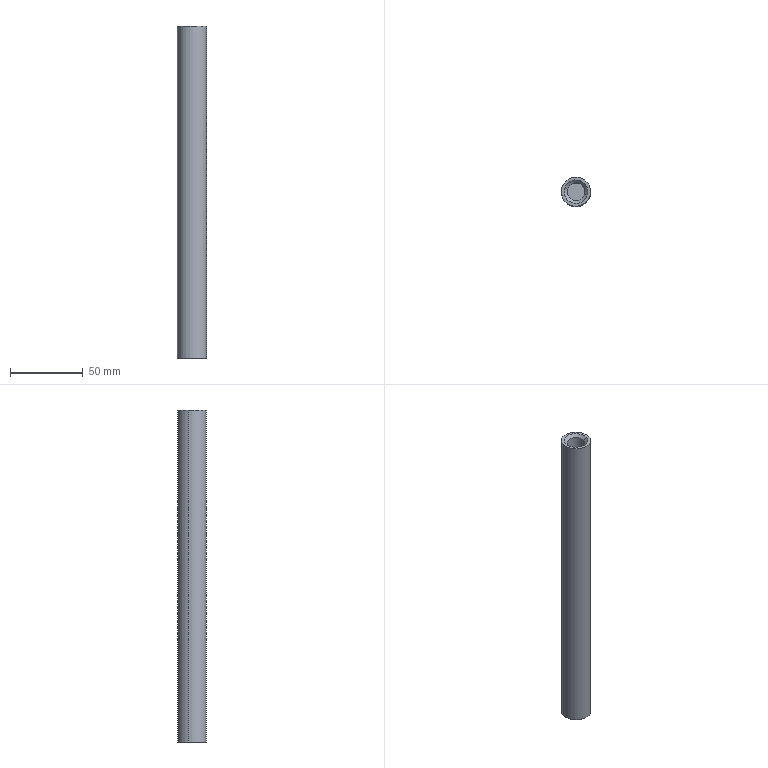Component | SolidWorks | BearingPressPartN-1 | 1 solid | 13 faces | box 20 x 20 x 228 mm | volume 58262 mm3 | cylinder 6 | cone 4 | plane 3 | commonest cylinder face diameters 14.5 x2 12.2 x2 20 x2
build123d program:
from build123d import *

# Parameters (mm, degrees)
SKETCH1_R                  = 10
BOSS_EXTRUDE1_DEPTH        = 228
SKETCH2_R                  = 6.1
CUT_EXTRUDE1_DEPTH         = 60
CHAMFER1_SIZE              = 2
M16X1_5_TAPPED_HOLE1_D     = 14.5
M16X1_5_TAPPED_HOLE1_DEPTH = 36.5
M16X1_5_TAPPED_HOLE1_TIP   = 4.356


with BuildPart() as part:
    # Sketch1 → Boss-Extrude1 (new body)
    with BuildSketch(Plane.XY):
        with Locations(Location((0, 0, 0), (0, 0, 180))):
            Circle(SKETCH1_R)
    extrude(amount=BOSS_EXTRUDE1_DEPTH)

    # Sketch2 → Cut-Extrude1 (cut)
    with BuildSketch(Plane(origin=(0, 0, 0), x_dir=(-1, 0, 0), z_dir=(0, 0, -1))):
        Circle(SKETCH2_R)
    extrude(amount=-CUT_EXTRUDE1_DEPTH, mode=Mode.SUBTRACT)

    # Chamfer1
    chamfer1_edges = [part.edges().sort_by_distance(p)[0] for p in [
        (6.1, 0, 0),
    ]]
    chamfer(chamfer1_edges, length=CHAMFER1_SIZE)

    # M16x1.5 Tapped Hole1
    with Locations(Plane.XY.offset(228)):
        with Locations((0, 0)):
            Hole(M16X1_5_TAPPED_HOLE1_D / 2, depth=M16X1_5_TAPPED_HOLE1_DEPTH)
            with Locations((0, 0, -(M16X1_5_TAPPED_HOLE1_DEPTH + M16X1_5_TAPPED_HOLE1_TIP / 2))):  # 118° drill point
                Cone(0, M16X1_5_TAPPED_HOLE1_D / 2, M16X1_5_TAPPED_HOLE1_TIP, mode=Mode.SUBTRACT)


solid = part.part

# Placed as in the assembly
solid = solid.moved(Location((447.676, 127.964, -266.218), (180, 0, 0)))
STEP:
#1=COLOUR_RGB('',0.7922,0.8196,0.9333);
#2=FILL_AREA_STYLE_COLOUR('',#1);
#3=FILL_AREA_STYLE('',(#2));
#4=SURFACE_STYLE_FILL_AREA(#3);
#5=SURFACE_SIDE_STYLE('',(#4));
#6=SURFACE_STYLE_USAGE(.BOTH.,#5);
#7=PRESENTATION_STYLE_ASSIGNMENT((#6));
#8=CARTESIAN_POINT('',(17.35,5.114,-18.02));
#9=VERTEX_POINT('',#8);
#10=CARTESIAN_POINT('',(17.9,4.962,-18.02));
#11=VERTEX_POINT('',#10);
#12=CARTESIAN_POINT('',(17.625,5.038,-18.02));
#13=DIRECTION('',(0.,-0.,-1.));
#14=DIRECTION('',(0.9638,-0.2665,0.));
#15=AXIS2_PLACEMENT_3D('',#12,#13,#14);
#16=CIRCLE('',#15,0.2854);
#17=EDGE_CURVE('',#9,#11,#16,.T.);
#18=ORIENTED_EDGE('',*,*,#17,.F.);
#19=CARTESIAN_POINT('',(17.35,5.114,-19.457));
#20=VERTEX_POINT('',#19);
#21=CARTESIAN_POINT('',(17.35,5.114,-19.457));
#22=DIRECTION('',(0.,-0.,-1.));
#23=VECTOR('',#22,39.37);
#24=LINE('',#21,#23);
#25=EDGE_CURVE('',#9,#20,#24,.T.);
#26=ORIENTED_EDGE('',*,*,#25,.T.);
#27=CARTESIAN_POINT('',(17.9,4.962,-19.457));
#28=VERTEX_POINT('',#27);
#29=CARTESIAN_POINT('',(17.625,5.038,-19.457));
#30=DIRECTION('',(0.,-0.,-1.));
#31=DIRECTION('',(0.9638,-0.2665,0.));
#32=AXIS2_PLACEMENT_3D('',#29,#30,#31);
#33=CIRCLE('',#32,0.2854);
#34=EDGE_CURVE('',#20,#28,#33,.T.);
#35=ORIENTED_EDGE('',*,*,#34,.T.);
#36=CARTESIAN_POINT('',(17.9,4.962,-19.457));
#37=DIRECTION('',(0.,-0.,-1.));
#38=VECTOR('',#37,39.37);
#39=LINE('',#36,#38);
#40=EDGE_CURVE('',#11,#28,#39,.T.);
#41=ORIENTED_EDGE('',*,*,#40,.F.);
#42=EDGE_LOOP('',(#18,#26,#35,#41));
#43=FACE_OUTER_BOUND('',#42,.T.);
#44=CARTESIAN_POINT('',(17.625,5.038,-19.457));
#45=DIRECTION('',(0.,-0.,-1.));
#46=DIRECTION('',(0.9638,-0.2665,0.));
#47=AXIS2_PLACEMENT_3D('',#44,#45,#46);
#48=CYLINDRICAL_SURFACE('',#47,0.2854);
#49=ADVANCED_FACE('',(#43),#48,.F.);
#50=CARTESIAN_POINT('',(17.625,5.038,-17.849));
#51=VERTEX_POINT('',#50);
#52=CARTESIAN_POINT('',(17.9,4.962,-18.02));
#53=DIRECTION('',(0.8262,-0.2284,-0.515));
#54=VECTOR('',#53,39.37);
#55=LINE('',#52,#54);
#56=EDGE_CURVE('',#51,#11,#55,.T.);
#57=ORIENTED_EDGE('',*,*,#56,.F.);
#58=CARTESIAN_POINT('',(17.35,5.114,-18.02));
#59=DIRECTION('',(-0.8262,0.2284,-0.515));
#60=VECTOR('',#59,39.37);
#61=LINE('',#58,#60);
#62=EDGE_CURVE('',#51,#9,#61,.T.);
#63=ORIENTED_EDGE('',*,*,#62,.T.);
#64=ORIENTED_EDGE('',*,*,#17,.T.);
#65=EDGE_LOOP('',(#57,#63,#64));
#66=FACE_OUTER_BOUND('',#65,.T.);
#67=CARTESIAN_POINT('',(17.625,5.038,-18.02));
#68=DIRECTION('',(0.,-0.,-1.));
#69=DIRECTION('',(0.9638,-0.2665,0.));
#70=AXIS2_PLACEMENT_3D('',#67,#68,#69);
#71=CONICAL_SURFACE('',#70,0.2854,1.03);
#72=ADVANCED_FACE('',(#66),#71,.F.);
#73=CARTESIAN_POINT('',(17.857,4.974,-10.56));
#74=VERTEX_POINT('',#73);
#75=CARTESIAN_POINT('',(17.394,5.102,-10.56));
#76=VERTEX_POINT('',#75);
#77=CARTESIAN_POINT('',(17.625,5.038,-10.56));
#78=DIRECTION('',(-0.,0.,1.));
#79=DIRECTION('',(0.9638,-0.2665,0.));
#80=AXIS2_PLACEMENT_3D('',#77,#78,#79);
#81=CIRCLE('',#80,0.2402);
#82=EDGE_CURVE('',#74,#76,#81,.T.);
#83=ORIENTED_EDGE('',*,*,#82,.F.);
#84=CARTESIAN_POINT('',(17.932,4.953,-10.481));
#85=VERTEX_POINT('',#84);
#86=CARTESIAN_POINT('',(17.857,4.974,-10.56));
#87=DIRECTION('',(0.6815,-0.1884,0.7071));
#88=VECTOR('',#87,39.37);
#89=LINE('',#86,#88);
#90=EDGE_CURVE('',#74,#85,#89,.T.);
#91=ORIENTED_EDGE('',*,*,#90,.T.);
#92=CARTESIAN_POINT('',(17.318,5.123,-10.481));
#93=VERTEX_POINT('',#92);
#94=CARTESIAN_POINT('',(17.625,5.038,-10.481));
#95=DIRECTION('',(0.,-0.,-1.));
#96=DIRECTION('',(0.9638,-0.2665,0.));
#97=AXIS2_PLACEMENT_3D('',#94,#95,#96);
#98=CIRCLE('',#97,0.3189);
#99=EDGE_CURVE('',#93,#85,#98,.T.);
#100=ORIENTED_EDGE('',*,*,#99,.F.);
#101=CARTESIAN_POINT('',(17.394,5.102,-10.56));
#102=DIRECTION('',(-0.6815,0.1884,0.7071));
#103=VECTOR('',#102,39.37);
#104=LINE('',#101,#103);
#105=EDGE_CURVE('',#76,#93,#104,.T.);
#106=ORIENTED_EDGE('',*,*,#105,.F.);
#107=EDGE_LOOP('',(#83,#91,#100,#106));
#108=FACE_OUTER_BOUND('',#107,.T.);
#109=CARTESIAN_POINT('',(17.625,5.038,-10.56));
#110=DIRECTION('',(-0.,0.,1.));
#111=DIRECTION('',(-0.9638,0.2665,0.));
#112=AXIS2_PLACEMENT_3D('',#109,#110,#111);
#113=CONICAL_SURFACE('',#112,0.2402,0.7854);
#114=ADVANCED_FACE('',(#108),#113,.F.);
#115=CARTESIAN_POINT('',(17.857,4.974,-12.843));
#116=VERTEX_POINT('',#115);
#117=CARTESIAN_POINT('',(17.394,5.102,-12.843));
#118=VERTEX_POINT('',#117);
#119=CARTESIAN_POINT('',(17.625,5.038,-12.843));
#120=DIRECTION('',(-0.,0.,1.));
#121=DIRECTION('',(-0.9638,0.2665,0.));
#122=AXIS2_PLACEMENT_3D('',#119,#120,#121);
#123=CIRCLE('',#122,0.2402);
#124=EDGE_CURVE('',#116,#118,#123,.T.);
#125=ORIENTED_EDGE('',*,*,#124,.F.);
#126=CARTESIAN_POINT('',(17.857,4.974,-12.843));
#127=DIRECTION('',(-0.,0.,1.));
#128=VECTOR('',#127,39.37);
#129=LINE('',#126,#128);
#130=EDGE_CURVE('',#116,#74,#129,.T.);
#131=ORIENTED_EDGE('',*,*,#130,.T.);
#132=ORIENTED_EDGE('',*,*,#82,.T.);
#133=CARTESIAN_POINT('',(17.394,5.102,-12.843));
#134=DIRECTION('',(-0.,0.,1.));
#135=VECTOR('',#134,39.37);
#136=LINE('',#133,#135);
#137=EDGE_CURVE('',#118,#76,#136,.T.);
#138=ORIENTED_EDGE('',*,*,#137,.F.);
#139=EDGE_LOOP('',(#125,#131,#132,#138));
#140=FACE_OUTER_BOUND('',#139,.T.);
#141=CARTESIAN_POINT('',(17.625,5.038,-12.843));
#142=DIRECTION('',(-0.,0.,1.));
#143=DIRECTION('',(-0.9638,0.2665,0.));
#144=AXIS2_PLACEMENT_3D('',#141,#142,#143);
#145=CYLINDRICAL_SURFACE('',#144,0.2402);
#146=ADVANCED_FACE('',(#140),#145,.F.);
#147=CARTESIAN_POINT('',(18.005,4.933,-19.457));
#148=VERTEX_POINT('',#147);
#149=CARTESIAN_POINT('',(17.246,5.143,-19.457));
#150=VERTEX_POINT('',#149);
#151=CARTESIAN_POINT('',(17.625,5.038,-19.457));
#152=DIRECTION('',(0.,-0.,-1.));
#153=DIRECTION('',(0.9638,-0.2665,0.));
#154=AXIS2_PLACEMENT_3D('',#151,#152,#153);
#155=CIRCLE('',#154,0.3937);
#156=EDGE_CURVE('',#148,#150,#155,.T.);
#157=ORIENTED_EDGE('',*,*,#156,.F.);
#158=CARTESIAN_POINT('',(18.005,4.933,-10.481));
#159=VERTEX_POINT('',#158);
#160=CARTESIAN_POINT('',(18.005,4.933,-19.457));
#161=DIRECTION('',(-0.,0.,1.));
#162=VECTOR('',#161,39.37);
#163=LINE('',#160,#162);
#164=EDGE_CURVE('',#148,#159,#163,.T.);
#165=ORIENTED_EDGE('',*,*,#164,.T.);
#166=CARTESIAN_POINT('',(17.246,5.143,-10.481));
#167=VERTEX_POINT('',#166);
#168=CARTESIAN_POINT('',(17.625,5.038,-10.481));
#169=DIRECTION('',(0.,-0.,-1.));
#170=DIRECTION('',(0.9638,-0.2665,0.));
#171=AXIS2_PLACEMENT_3D('',#168,#169,#170);
#172=CIRCLE('',#171,0.3937);
#173=EDGE_CURVE('',#159,#167,#172,.T.);
#174=ORIENTED_EDGE('',*,*,#173,.T.);
#175=CARTESIAN_POINT('',(17.246,5.143,-19.457));
#176=DIRECTION('',(-0.,0.,1.));
#177=VECTOR('',#176,39.37);
#178=LINE('',#175,#177);
#179=EDGE_CURVE('',#150,#167,#178,.T.);
#180=ORIENTED_EDGE('',*,*,#179,.F.);
#181=EDGE_LOOP('',(#157,#165,#174,#180));
#182=FACE_OUTER_BOUND('',#181,.T.);
#183=CARTESIAN_POINT('',(17.625,5.038,-19.457));
#184=DIRECTION('',(-0.,0.,1.));
#185=DIRECTION('',(-0.9638,0.2665,0.));
#186=AXIS2_PLACEMENT_3D('',#183,#184,#185);
#187=CYLINDRICAL_SURFACE('',#186,0.3937);
#188=ADVANCED_FACE('',(#182),#187,.T.);
#189=ORIENTED_EDGE('',*,*,#164,.F.);
#190=CARTESIAN_POINT('',(17.625,5.038,-19.457));
#191=DIRECTION('',(0.,-0.,-1.));
#192=DIRECTION('',(0.9638,-0.2665,0.));
#193=AXIS2_PLACEMENT_3D('',#190,#191,#192);
#194=CIRCLE('',#193,0.3937);
#195=EDGE_CURVE('',#150,#148,#194,.T.);
#196=ORIENTED_EDGE('',*,*,#195,.F.);
#197=ORIENTED_EDGE('',*,*,#179,.T.);
#198=CARTESIAN_POINT('',(17.625,5.038,-10.481));
#199=DIRECTION('',(0.,-0.,-1.));
#200=DIRECTION('',(0.9638,-0.2665,0.));
#201=AXIS2_PLACEMENT_3D('',#198,#199,#200);
#202=CIRCLE('',#201,0.3937);
#203=EDGE_CURVE('',#167,#159,#202,.T.);
#204=ORIENTED_EDGE('',*,*,#203,.T.);
#205=EDGE_LOOP('',(#189,#196,#197,#204));
#206=FACE_OUTER_BOUND('',#205,.T.);
#207=CARTESIAN_POINT('',(17.625,5.038,-19.457));
#208=DIRECTION('',(-0.,0.,1.));
#209=DIRECTION('',(-0.9638,0.2665,0.));
#210=AXIS2_PLACEMENT_3D('',#207,#208,#209);
#211=CYLINDRICAL_SURFACE('',#210,0.3937);
#212=ADVANCED_FACE('',(#206),#211,.T.);
#213=CARTESIAN_POINT('',(17.625,5.038,-19.457));
#214=DIRECTION('',(0.,-0.,-1.));
#215=DIRECTION('',(0.9638,-0.2665,0.));
#216=AXIS2_PLACEMENT_3D('',#213,#214,#215);
#217=CIRCLE('',#216,0.2854);
#218=EDGE_CURVE('',#28,#20,#217,.T.);
#219=ORIENTED_EDGE('',*,*,#218,.F.);
#220=ORIENTED_EDGE('',*,*,#34,.F.);
#221=EDGE_LOOP('',(#219,#220));
#222=FACE_BOUND('',#221,.T.);
#223=ORIENTED_EDGE('',*,*,#195,.T.);
#224=ORIENTED_EDGE('',*,*,#156,.T.);
#225=EDGE_LOOP('',(#223,#224));
#226=FACE_OUTER_BOUND('',#225,.T.);
#227=CARTESIAN_POINT('',(17.625,5.038,-19.457));
#228=DIRECTION('',(0.,-0.,-1.));
#229=DIRECTION('',(0.9638,-0.2665,0.));
#230=AXIS2_PLACEMENT_3D('',#227,#228,#229);
#231=PLANE('',#230);
#232=ADVANCED_FACE('',(#222,#226),#231,.T.);
#233=ORIENTED_EDGE('',*,*,#99,.T.);
#234=CARTESIAN_POINT('',(17.625,5.038,-10.481));
#235=DIRECTION('',(0.,-0.,-1.));
#236=DIRECTION('',(0.9638,-0.2665,0.));
#237=AXIS2_PLACEMENT_3D('',#234,#235,#236);
#238=CIRCLE('',#237,0.3189);
#239=EDGE_CURVE('',#85,#93,#238,.T.);
#240=ORIENTED_EDGE('',*,*,#239,.T.);
#241=EDGE_LOOP('',(#233,#240));
#242=FACE_BOUND('',#241,.T.);
#243=ORIENTED_EDGE('',*,*,#203,.F.);
#244=ORIENTED_EDGE('',*,*,#173,.F.);
#245=EDGE_LOOP('',(#243,#244));
#246=FACE_OUTER_BOUND('',#245,.T.);
#247=CARTESIAN_POINT('',(17.625,5.038,-10.481));
#248=DIRECTION('',(0.,-0.,-1.));
#249=DIRECTION('',(0.9638,-0.2665,0.));
#250=AXIS2_PLACEMENT_3D('',#247,#248,#249);
#251=PLANE('',#250);
#252=ADVANCED_FACE('',(#242,#246),#251,.F.);
#253=ORIENTED_EDGE('',*,*,#130,.F.);
#254=CARTESIAN_POINT('',(17.625,5.038,-12.843));
#255=DIRECTION('',(-0.,0.,1.));
#256=DIRECTION('',(-0.9638,0.2665,0.));
#257=AXIS2_PLACEMENT_3D('',#254,#255,#256);
#258=CIRCLE('',#257,0.2402);
#259=EDGE_CURVE('',#118,#116,#258,.T.);
#260=ORIENTED_EDGE('',*,*,#259,.F.);
#261=ORIENTED_EDGE('',*,*,#137,.T.);
#262=CARTESIAN_POINT('',(17.625,5.038,-10.56));
#263=DIRECTION('',(-0.,0.,1.));
#264=DIRECTION('',(0.9638,-0.2665,0.));
#265=AXIS2_PLACEMENT_3D('',#262,#263,#264);
#266=CIRCLE('',#265,0.2402);
#267=EDGE_CURVE('',#76,#74,#266,.T.);
#268=ORIENTED_EDGE('',*,*,#267,.T.);
#269=EDGE_LOOP('',(#253,#260,#261,#268));
#270=FACE_OUTER_BOUND('',#269,.T.);
#271=CARTESIAN_POINT('',(17.625,5.038,-12.843));
#272=DIRECTION('',(-0.,0.,1.));
#273=DIRECTION('',(-0.9638,0.2665,0.));
#274=AXIS2_PLACEMENT_3D('',#271,#272,#273);
#275=CYLINDRICAL_SURFACE('',#274,0.2402);
#276=ADVANCED_FACE('',(#270),#275,.F.);
#277=ORIENTED_EDGE('',*,*,#259,.T.);
#278=ORIENTED_EDGE('',*,*,#124,.T.);
#279=EDGE_LOOP('',(#277,#278));
#280=FACE_OUTER_BOUND('',#279,.T.);
#281=CARTESIAN_POINT('',(17.625,5.038,-12.843));
#282=DIRECTION('',(-0.,0.,1.));
#283=DIRECTION('',(-0.9638,0.2665,-0.));
#284=AXIS2_PLACEMENT_3D('',#281,#282,#283);
#285=PLANE('',#284);
#286=ADVANCED_FACE('',(#280),#285,.T.);
#287=ORIENTED_EDGE('',*,*,#90,.F.);
#288=ORIENTED_EDGE('',*,*,#267,.F.);
#289=ORIENTED_EDGE('',*,*,#105,.T.);
#290=ORIENTED_EDGE('',*,*,#239,.F.);
#291=EDGE_LOOP('',(#287,#288,#289,#290));
#292=FACE_OUTER_BOUND('',#291,.T.);
#293=CARTESIAN_POINT('',(17.625,5.038,-10.56));
#294=DIRECTION('',(-0.,0.,1.));
#295=DIRECTION('',(-0.9638,0.2665,0.));
#296=AXIS2_PLACEMENT_3D('',#293,#294,#295);
#297=CONICAL_SURFACE('',#296,0.2402,0.7854);
#298=ADVANCED_FACE('',(#292),#297,.F.);
#299=ORIENTED_EDGE('',*,*,#62,.F.);
#300=ORIENTED_EDGE('',*,*,#56,.T.);
#301=CARTESIAN_POINT('',(17.625,5.038,-18.02));
#302=DIRECTION('',(0.,-0.,-1.));
#303=DIRECTION('',(0.9638,-0.2665,0.));
#304=AXIS2_PLACEMENT_3D('',#301,#302,#303);
#305=CIRCLE('',#304,0.2854);
#306=EDGE_CURVE('',#11,#9,#305,.T.);
#307=ORIENTED_EDGE('',*,*,#306,.T.);
#308=EDGE_LOOP('',(#299,#300,#307));
#309=FACE_OUTER_BOUND('',#308,.T.);
#310=CARTESIAN_POINT('',(17.625,5.038,-18.02));
#311=DIRECTION('',(0.,-0.,-1.));
#312=DIRECTION('',(0.9638,-0.2665,0.));
#313=AXIS2_PLACEMENT_3D('',#310,#311,#312);
#314=CONICAL_SURFACE('',#313,0.2854,1.03);
#315=ADVANCED_FACE('',(#309),#314,.F.);
#316=ORIENTED_EDGE('',*,*,#25,.F.);
#317=ORIENTED_EDGE('',*,*,#306,.F.);
#318=ORIENTED_EDGE('',*,*,#40,.T.);
#319=ORIENTED_EDGE('',*,*,#218,.T.);
#320=EDGE_LOOP('',(#316,#317,#318,#319));
#321=FACE_OUTER_BOUND('',#320,.T.);
#322=CARTESIAN_POINT('',(17.625,5.038,-19.457));
#323=DIRECTION('',(0.,-0.,-1.));
#324=DIRECTION('',(0.9638,-0.2665,0.));
#325=AXIS2_PLACEMENT_3D('',#322,#323,#324);
#326=CYLINDRICAL_SURFACE('',#325,0.2854);
#327=ADVANCED_FACE('',(#321),#326,.F.);
#328=CLOSED_SHELL('',(#49,#72,#114,#146,#188,#212,#232,#252,#276,#286,#298,#315,#327));
#329=MANIFOLD_SOLID_BREP('',#328);
#330=STYLED_ITEM('',(#7),#329);
#331=(LENGTH_UNIT()NAMED_UNIT(*)SI_UNIT($,.METRE.));
#332=LENGTH_MEASURE_WITH_UNIT(LENGTH_MEASURE(0.0254),#331);
#333=DIMENSIONAL_EXPONENTS(1.,0.,0.,0.,0.,0.,0.);
#334=(CONVERSION_BASED_UNIT('',#332)LENGTH_UNIT()NAMED_UNIT(#333));
#335=UNCERTAINTY_MEASURE_WITH_UNIT(LENGTH_MEASURE(0.00001),#334,'','');
#336=(NAMED_UNIT(*)PLANE_ANGLE_UNIT()SI_UNIT($,.RADIAN.));
#337=(NAMED_UNIT(*)SI_UNIT($,.STERADIAN.)SOLID_ANGLE_UNIT());
#338=(GEOMETRIC_REPRESENTATION_CONTEXT(3)GLOBAL_UNCERTAINTY_ASSIGNED_CONTEXT((#335))GLOBAL_UNIT_ASSIGNED_CONTEXT((#334,#336,#337))REPRESENTATION_CONTEXT('',''));
#339=MECHANICAL_DESIGN_GEOMETRIC_PRESENTATION_REPRESENTATION('',(#330),#338);
#340=PRESENTATION_LAYER_ASSIGNMENT('','',(#330));
#341=CARTESIAN_POINT('',(0.,0.,0.));
#342=DIRECTION('',(0.,0.,1.));
#343=DIRECTION('',(1.,0.,0.));
#344=AXIS2_PLACEMENT_3D('',#341,#342,#343);
#345=(LENGTH_UNIT()NAMED_UNIT(*)SI_UNIT($,.METRE.));
#346=LENGTH_MEASURE_WITH_UNIT(LENGTH_MEASURE(0.0254),#345);
#347=DIMENSIONAL_EXPONENTS(1.,0.,0.,0.,0.,0.,0.);
#348=(CONVERSION_BASED_UNIT('',#346)LENGTH_UNIT()NAMED_UNIT(#347));
#349=UNCERTAINTY_MEASURE_WITH_UNIT(LENGTH_MEASURE(0.00001),#348,'','');
#350=(NAMED_UNIT(*)PLANE_ANGLE_UNIT()SI_UNIT($,.RADIAN.));
#351=(NAMED_UNIT(*)SI_UNIT($,.STERADIAN.)SOLID_ANGLE_UNIT());
#352=(GEOMETRIC_REPRESENTATION_CONTEXT(3)GLOBAL_UNCERTAINTY_ASSIGNED_CONTEXT((#349))GLOBAL_UNIT_ASSIGNED_CONTEXT((#348,#350,#351))REPRESENTATION_CONTEXT('',''));
#353=ADVANCED_BREP_SHAPE_REPRESENTATION('',(#329,#344),#352);